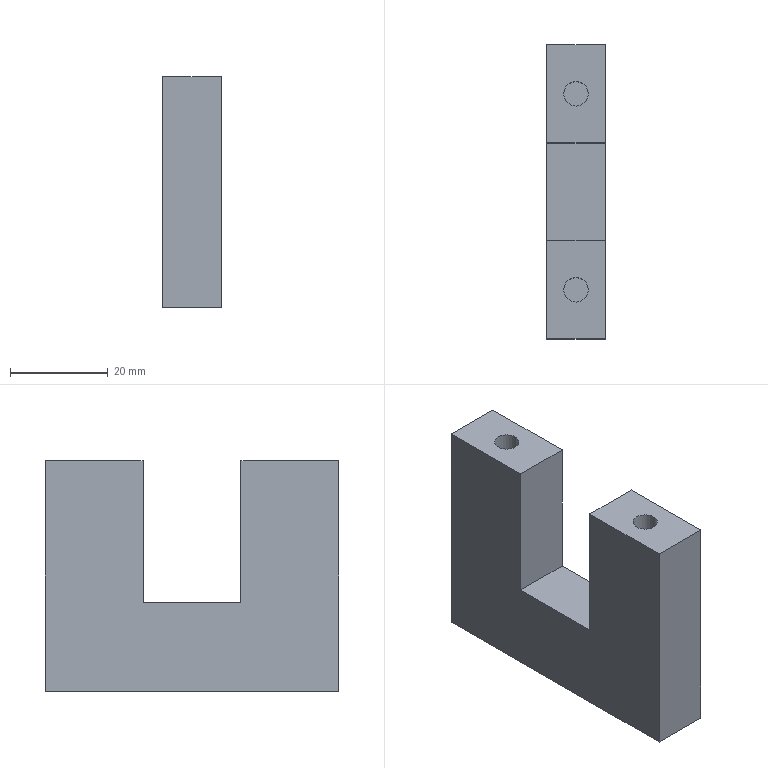Component | NX | U_PLATE | 1 solid | 22 faces | volume 24995 mm3 | plane 16 | cylinder 6 | commonest cylinder face diameters 5 x6